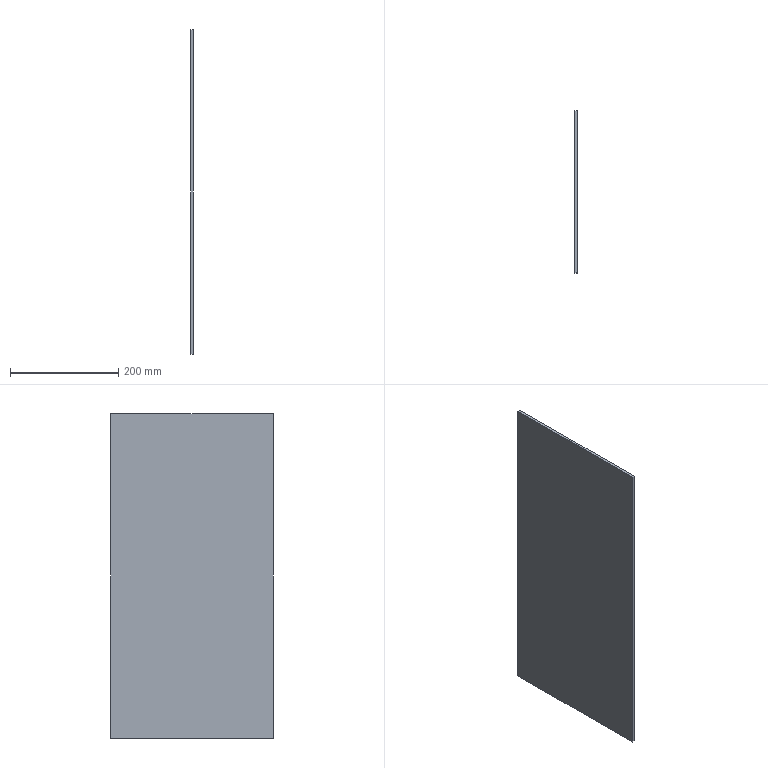Component | SolidWorks | CoverPlate1-1 | 1 solid | 6 faces | box 5 x 300 x 600 mm | volume 900000 mm3 | plane 6
build123d program:
from build123d import *

# Parameters (mm, degrees)
SKETCH1_W      = 300
SKETCH1_H      = 600
EXTRUDE1_DEPTH = 5


with BuildPart() as part:
    # Sketch1 → Extrude1 (new body)
    with BuildSketch(Plane.XY):
        Rectangle(SKETCH1_W, SKETCH1_H)
    extrude(amount=EXTRUDE1_DEPTH)


solid = part.part

# Placed as in the assembly
solid = solid.moved(Location((-300, -10, 280), (90, -90, 0)))
STEP:
#1=COLOUR_RGB('',0.7922,0.8196,0.9333);
#2=FILL_AREA_STYLE_COLOUR('',#1);
#3=FILL_AREA_STYLE('',(#2));
#4=SURFACE_STYLE_FILL_AREA(#3);
#5=SURFACE_SIDE_STYLE('',(#4));
#6=SURFACE_STYLE_USAGE(.BOTH.,#5);
#7=PRESENTATION_STYLE_ASSIGNMENT((#6));
#8=CARTESIAN_POINT('',(-12.008,5.512,-0.7874));
#9=VERTEX_POINT('',#8);
#10=CARTESIAN_POINT('',(-12.008,5.512,22.835));
#11=VERTEX_POINT('',#10);
#12=CARTESIAN_POINT('',(-12.008,5.512,22.835));
#13=DIRECTION('',(0.,-0.,1.));
#14=VECTOR('',#13,39.37);
#15=LINE('',#12,#14);
#16=EDGE_CURVE('',#9,#11,#15,.T.);
#17=ORIENTED_EDGE('',*,*,#16,.T.);
#18=CARTESIAN_POINT('',(-11.811,5.512,22.835));
#19=VERTEX_POINT('',#18);
#20=CARTESIAN_POINT('',(-11.811,5.512,22.835));
#21=DIRECTION('',(-1.,-0.,0.));
#22=VECTOR('',#21,39.37);
#23=LINE('',#20,#22);
#24=EDGE_CURVE('',#19,#11,#23,.T.);
#25=ORIENTED_EDGE('',*,*,#24,.F.);
#26=CARTESIAN_POINT('',(-11.811,5.512,-0.7874));
#27=VERTEX_POINT('',#26);
#28=CARTESIAN_POINT('',(-11.811,5.512,22.835));
#29=DIRECTION('',(0.,-0.,1.));
#30=VECTOR('',#29,39.37);
#31=LINE('',#28,#30);
#32=EDGE_CURVE('',#27,#19,#31,.T.);
#33=ORIENTED_EDGE('',*,*,#32,.F.);
#34=CARTESIAN_POINT('',(-11.811,5.512,-0.7874));
#35=DIRECTION('',(-1.,-0.,0.));
#36=VECTOR('',#35,39.37);
#37=LINE('',#34,#36);
#38=EDGE_CURVE('',#27,#9,#37,.T.);
#39=ORIENTED_EDGE('',*,*,#38,.T.);
#40=EDGE_LOOP('',(#17,#25,#33,#39));
#41=FACE_OUTER_BOUND('',#40,.T.);
#42=CARTESIAN_POINT('',(-11.811,5.512,22.835));
#43=DIRECTION('',(0.,-1.,-0.));
#44=DIRECTION('',(-0.,0.,-1.));
#45=AXIS2_PLACEMENT_3D('',#42,#43,#44);
#46=PLANE('',#45);
#47=ADVANCED_FACE('',(#41),#46,.F.);
#48=CARTESIAN_POINT('',(-12.008,-6.299,22.835));
#49=VERTEX_POINT('',#48);
#50=CARTESIAN_POINT('',(-12.008,-6.299,22.835));
#51=DIRECTION('',(0.,-1.,0.));
#52=VECTOR('',#51,39.37);
#53=LINE('',#50,#52);
#54=EDGE_CURVE('',#11,#49,#53,.T.);
#55=ORIENTED_EDGE('',*,*,#54,.T.);
#56=CARTESIAN_POINT('',(-11.811,-6.299,22.835));
#57=VERTEX_POINT('',#56);
#58=CARTESIAN_POINT('',(-11.811,-6.299,22.835));
#59=DIRECTION('',(-1.,-0.,0.));
#60=VECTOR('',#59,39.37);
#61=LINE('',#58,#60);
#62=EDGE_CURVE('',#57,#49,#61,.T.);
#63=ORIENTED_EDGE('',*,*,#62,.F.);
#64=CARTESIAN_POINT('',(-11.811,-6.299,22.835));
#65=DIRECTION('',(0.,-1.,0.));
#66=VECTOR('',#65,39.37);
#67=LINE('',#64,#66);
#68=EDGE_CURVE('',#19,#57,#67,.T.);
#69=ORIENTED_EDGE('',*,*,#68,.F.);
#70=ORIENTED_EDGE('',*,*,#24,.T.);
#71=EDGE_LOOP('',(#55,#63,#69,#70));
#72=FACE_OUTER_BOUND('',#71,.T.);
#73=CARTESIAN_POINT('',(-11.811,-6.299,22.835));
#74=DIRECTION('',(-0.,-0.,-1.));
#75=DIRECTION('',(-1.,-0.,0.));
#76=AXIS2_PLACEMENT_3D('',#73,#74,#75);
#77=PLANE('',#76);
#78=ADVANCED_FACE('',(#72),#77,.F.);
#79=CARTESIAN_POINT('',(-12.008,-6.299,-0.7874));
#80=VERTEX_POINT('',#79);
#81=CARTESIAN_POINT('',(-12.008,-6.299,22.835));
#82=DIRECTION('',(-0.,0.,-1.));
#83=VECTOR('',#82,39.37);
#84=LINE('',#81,#83);
#85=EDGE_CURVE('',#49,#80,#84,.T.);
#86=ORIENTED_EDGE('',*,*,#85,.T.);
#87=CARTESIAN_POINT('',(-11.811,-6.299,-0.7874));
#88=VERTEX_POINT('',#87);
#89=CARTESIAN_POINT('',(-11.811,-6.299,-0.7874));
#90=DIRECTION('',(-1.,-0.,0.));
#91=VECTOR('',#90,39.37);
#92=LINE('',#89,#91);
#93=EDGE_CURVE('',#88,#80,#92,.T.);
#94=ORIENTED_EDGE('',*,*,#93,.F.);
#95=CARTESIAN_POINT('',(-11.811,-6.299,22.835));
#96=DIRECTION('',(-0.,0.,-1.));
#97=VECTOR('',#96,39.37);
#98=LINE('',#95,#97);
#99=EDGE_CURVE('',#57,#88,#98,.T.);
#100=ORIENTED_EDGE('',*,*,#99,.F.);
#101=ORIENTED_EDGE('',*,*,#62,.T.);
#102=EDGE_LOOP('',(#86,#94,#100,#101));
#103=FACE_OUTER_BOUND('',#102,.T.);
#104=CARTESIAN_POINT('',(-11.811,-6.299,22.835));
#105=DIRECTION('',(-0.,1.,0.));
#106=DIRECTION('',(0.,-0.,1.));
#107=AXIS2_PLACEMENT_3D('',#104,#105,#106);
#108=PLANE('',#107);
#109=ADVANCED_FACE('',(#103),#108,.F.);
#110=CARTESIAN_POINT('',(-12.008,-6.299,-0.7874));
#111=DIRECTION('',(-0.,1.,-0.));
#112=VECTOR('',#111,39.37);
#113=LINE('',#110,#112);
#114=EDGE_CURVE('',#80,#9,#113,.T.);
#115=ORIENTED_EDGE('',*,*,#114,.T.);
#116=ORIENTED_EDGE('',*,*,#38,.F.);
#117=CARTESIAN_POINT('',(-11.811,-6.299,-0.7874));
#118=DIRECTION('',(-0.,1.,-0.));
#119=VECTOR('',#118,39.37);
#120=LINE('',#117,#119);
#121=EDGE_CURVE('',#88,#27,#120,.T.);
#122=ORIENTED_EDGE('',*,*,#121,.F.);
#123=ORIENTED_EDGE('',*,*,#93,.T.);
#124=EDGE_LOOP('',(#115,#116,#122,#123));
#125=FACE_OUTER_BOUND('',#124,.T.);
#126=CARTESIAN_POINT('',(-11.811,-6.299,-0.7874));
#127=DIRECTION('',(0.,0.,1.));
#128=DIRECTION('',(1.,0.,-0.));
#129=AXIS2_PLACEMENT_3D('',#126,#127,#128);
#130=PLANE('',#129);
#131=ADVANCED_FACE('',(#125),#130,.F.);
#132=ORIENTED_EDGE('',*,*,#32,.T.);
#133=ORIENTED_EDGE('',*,*,#68,.T.);
#134=ORIENTED_EDGE('',*,*,#99,.T.);
#135=ORIENTED_EDGE('',*,*,#121,.T.);
#136=EDGE_LOOP('',(#132,#133,#134,#135));
#137=FACE_OUTER_BOUND('',#136,.T.);
#138=CARTESIAN_POINT('',(-11.811,-0.3937,11.024));
#139=DIRECTION('',(1.,0.,-0.));
#140=DIRECTION('',(-0.,1.,-0.));
#141=AXIS2_PLACEMENT_3D('',#138,#139,#140);
#142=PLANE('',#141);
#143=ADVANCED_FACE('',(#137),#142,.T.);
#144=ORIENTED_EDGE('',*,*,#16,.F.);
#145=ORIENTED_EDGE('',*,*,#114,.F.);
#146=ORIENTED_EDGE('',*,*,#85,.F.);
#147=ORIENTED_EDGE('',*,*,#54,.F.);
#148=EDGE_LOOP('',(#144,#145,#146,#147));
#149=FACE_OUTER_BOUND('',#148,.T.);
#150=CARTESIAN_POINT('',(-12.008,-0.3937,11.024));
#151=DIRECTION('',(1.,0.,-0.));
#152=DIRECTION('',(-0.,1.,-0.));
#153=AXIS2_PLACEMENT_3D('',#150,#151,#152);
#154=PLANE('',#153);
#155=ADVANCED_FACE('',(#149),#154,.F.);
#156=CLOSED_SHELL('',(#47,#78,#109,#131,#143,#155));
#157=MANIFOLD_SOLID_BREP('',#156);
#158=STYLED_ITEM('',(#7),#157);
#159=PRESENTATION_LAYER_ASSIGNMENT('','',(#158));
#160=(LENGTH_UNIT()NAMED_UNIT(*)SI_UNIT($,.METRE.));
#161=LENGTH_MEASURE_WITH_UNIT(LENGTH_MEASURE(0.0254),#160);
#162=DIMENSIONAL_EXPONENTS(1.,0.,0.,0.,0.,0.,0.);
#163=(CONVERSION_BASED_UNIT('',#161)LENGTH_UNIT()NAMED_UNIT(#162));
#164=UNCERTAINTY_MEASURE_WITH_UNIT(LENGTH_MEASURE(0.00001),#163,'','');
#165=(NAMED_UNIT(*)PLANE_ANGLE_UNIT()SI_UNIT($,.RADIAN.));
#166=(NAMED_UNIT(*)SI_UNIT($,.STERADIAN.)SOLID_ANGLE_UNIT());
#167=(GEOMETRIC_REPRESENTATION_CONTEXT(3)GLOBAL_UNCERTAINTY_ASSIGNED_CONTEXT((#164))GLOBAL_UNIT_ASSIGNED_CONTEXT((#163,#165,#166))REPRESENTATION_CONTEXT('',''));
#168=MECHANICAL_DESIGN_GEOMETRIC_PRESENTATION_REPRESENTATION('',(#158),#167);
#169=CARTESIAN_POINT('',(0.,0.,0.));
#170=DIRECTION('',(0.,0.,1.));
#171=DIRECTION('',(1.,0.,0.));
#172=AXIS2_PLACEMENT_3D('',#169,#170,#171);
#173=(LENGTH_UNIT()NAMED_UNIT(*)SI_UNIT($,.METRE.));
#174=LENGTH_MEASURE_WITH_UNIT(LENGTH_MEASURE(0.0254),#173);
#175=DIMENSIONAL_EXPONENTS(1.,0.,0.,0.,0.,0.,0.);
#176=(CONVERSION_BASED_UNIT('',#174)LENGTH_UNIT()NAMED_UNIT(#175));
#177=UNCERTAINTY_MEASURE_WITH_UNIT(LENGTH_MEASURE(0.00001),#176,'','');
#178=(NAMED_UNIT(*)PLANE_ANGLE_UNIT()SI_UNIT($,.RADIAN.));
#179=(NAMED_UNIT(*)SI_UNIT($,.STERADIAN.)SOLID_ANGLE_UNIT());
#180=(GEOMETRIC_REPRESENTATION_CONTEXT(3)GLOBAL_UNCERTAINTY_ASSIGNED_CONTEXT((#177))GLOBAL_UNIT_ASSIGNED_CONTEXT((#176,#178,#179))REPRESENTATION_CONTEXT('',''));
#181=ADVANCED_BREP_SHAPE_REPRESENTATION('',(#157,#172),#180);